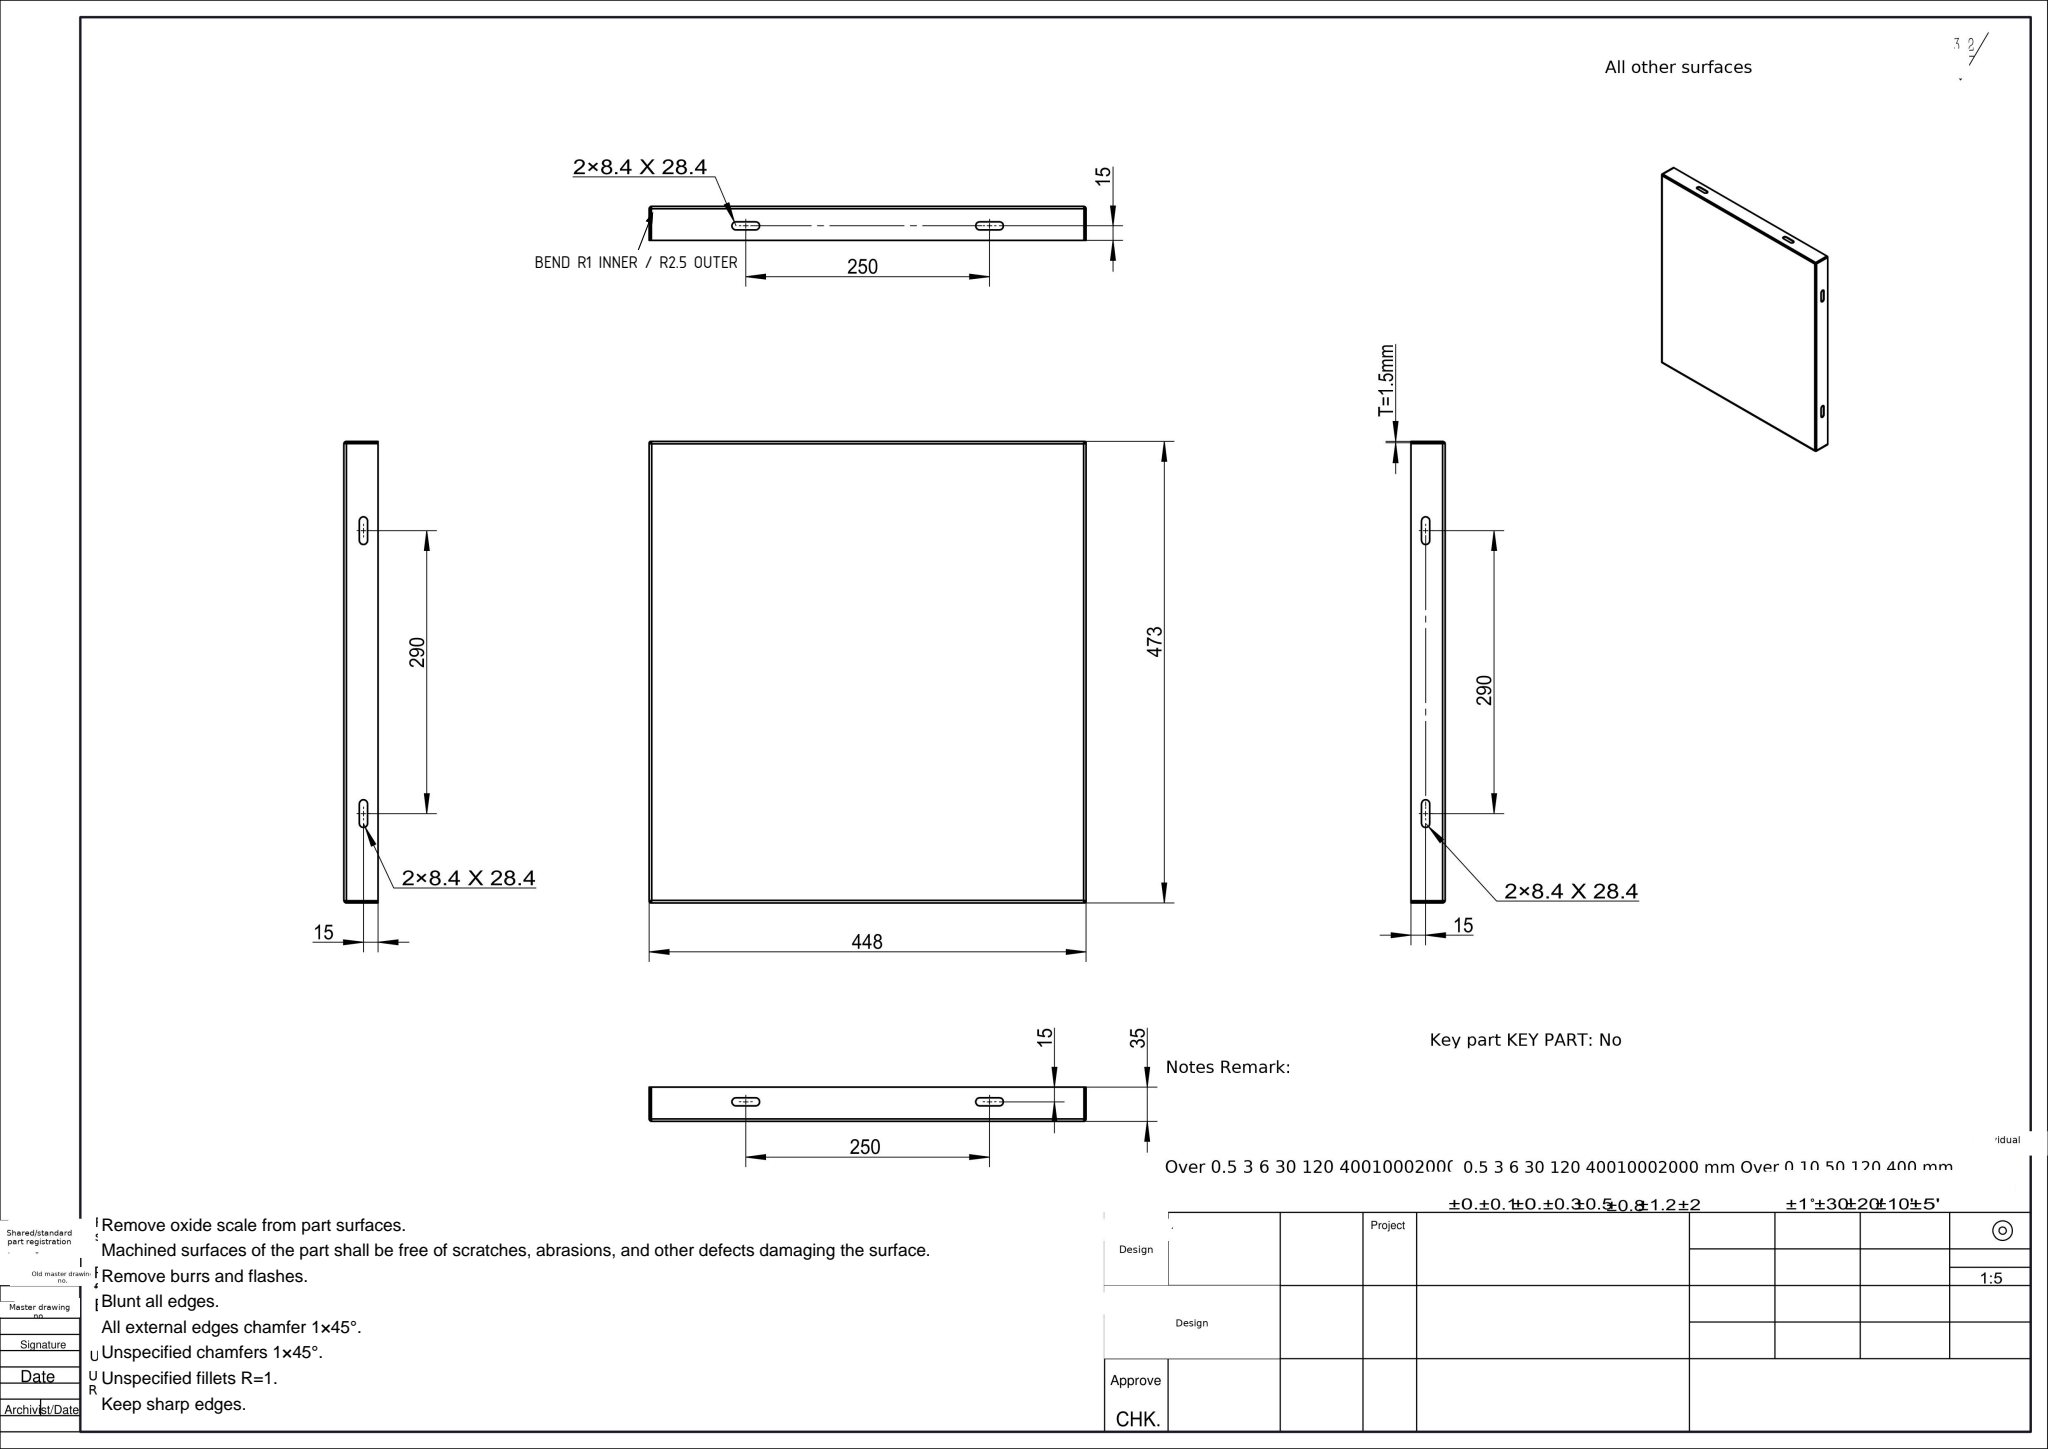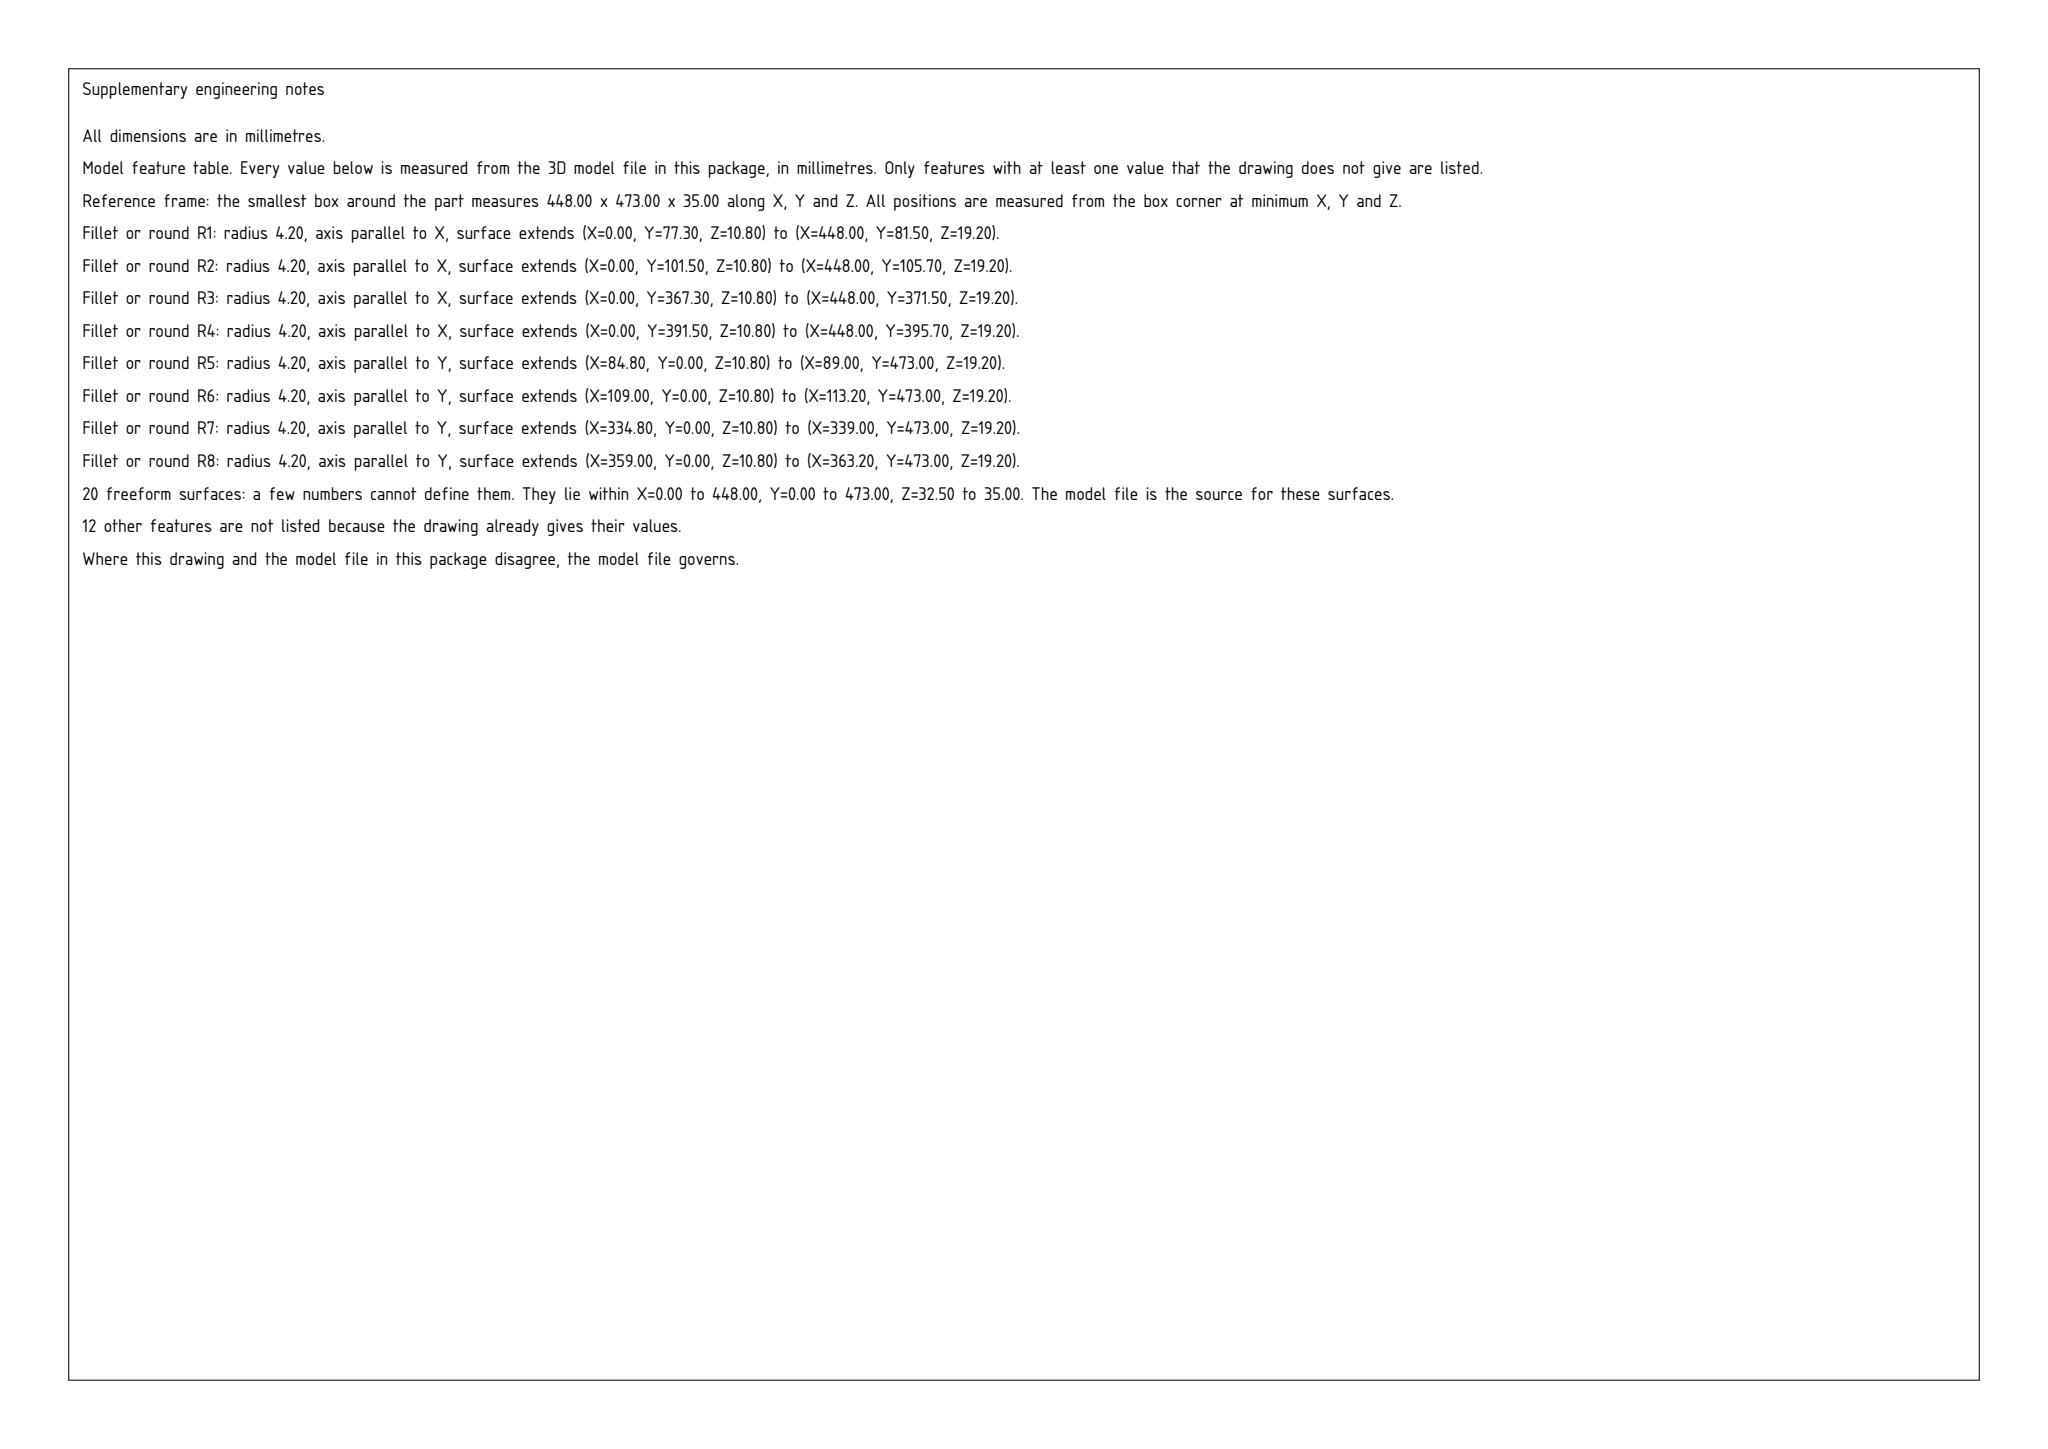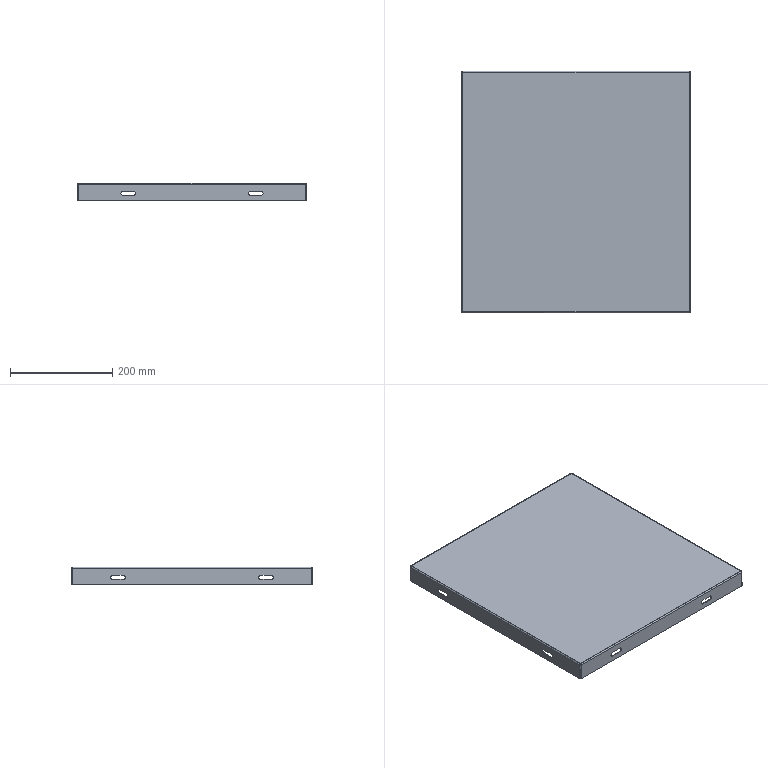Part | SolidWorks | mm | 1 solid | 98 faces | box 448 x 473 x 35 mm | volume 405300 mm3 | plane 50 | cylinder 28 | spline 20 | commonest cylinder face diameters 8.4 x16 5 x4 2 x4 3 x4
Drawing notes:
Flange bend radii: inner R1 (Ø2) and outer R2.5 (Ø5) at all four bend lines, radius centers 2.5 in from each outer face at Z=32.5, sheet T=1.5. | from the solid: cylinders dia 2.0 and 5.0, axes x and y, positions at 2.5/445.5 and 2.5/470.5 with Z=32.5, lengths 443.59/468.59
GEN TOL RANGES mm: 0.5-3,3-6,6-30,30-120,120-400,400-1000,1000-4000 | from the solid: GB/T 1804-2000-m table header on sheet; part sizes 448x473x35 fall in 400-1000 range
LINEAR GEN TOL m: ±0.1/±0.1/±0.2/±0.3/±0.5/±0.8/±1.2/±2 | from the solid: GB/T 1804-2000-m linear values per listed size ranges; 448/473 use ±0.8
ANG TOL m: <10 ±1°; -50 ±30'; -120 ±20'; -400 ±10'; >400 ±5' | from the solid: GB/T 1804-2000-m angular values per short-side length ranges 0-10-50-120-400 mm